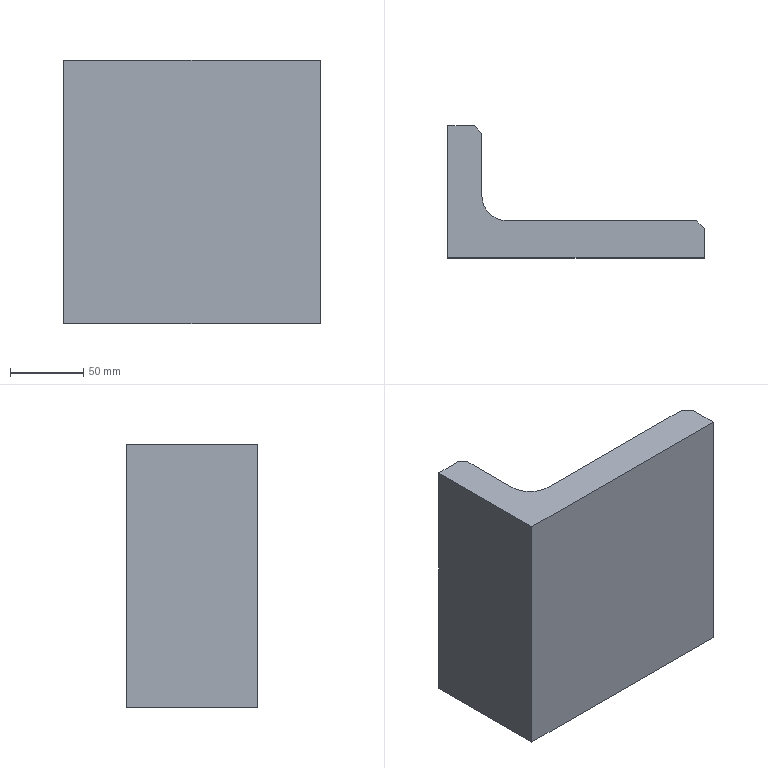Component | SolidWorks | L-Plate-1 | 1 solid | 20 faces | box 175 x 90 x 180 mm | volume 513210 mm3 | plane 18 | cylinder 2 | commonest cylinder face diameters 35.105 x2
build123d program:
from build123d import *

# Parameters (mm, degrees)
BOSS_EXTRUDE1_DEPTH = 90
BOSS_EXTRUDE3_DEPTH = 8
CHAMFER1_SIZE       = 5


with BuildPart() as part:
    # Sketch1 → Boss-Extrude1 (new, symmetric)
    with BuildSketch(Plane.XY):
        Polygon((0, 90), (0, 0), (-175, 0), (-175, 10), (-10, 10), (-10, 90), align=None)
    extrude(amount=BOSS_EXTRUDE1_DEPTH, both=True)

    # Sketch3 → Boss-Extrude3 (add)
    with BuildSketch(Plane(origin=(0, 0, -90), x_dir=(-1, 0, 0), z_dir=(0, 0, -1))):
        with BuildLine():
            Line((10, 90), (23.172, 90))
            Line((23.172, 90), (23.172, 42.657))
            ThreePointArc((23.172, 42.657), (28.312, 30.246), (40.724, 25.105))
            Line((40.724, 25.105), (175, 25.105))
            Line((175, 25.105), (175, 10))
            Line((175, 10), (10, 10))
            Line((10, 10), (10, 90))
        make_face()
    boss_extrude3 = extrude(amount=-BOSS_EXTRUDE3_DEPTH)

    # Mirror1: Boss-Extrude3 across plane
    add(boss_extrude3.mirror(Plane.XY))

    # Chamfer1
    chamfer1_edges = [part.edges().sort_by_distance(p)[0] for p in [
        (-23.172, 90, -86),
        (-175, 25.105, -86),
        (-175, 25.105, 86),
        (-23.172, 90, 86),
    ]]
    chamfer(chamfer1_edges, length=CHAMFER1_SIZE)


solid = part.part

# Placed as in the assembly
solid = solid.moved(Location((95.398, 325.813, 100), (-180, 0, 180)))
STEP:
#1=COLOUR_RGB('',0.7922,0.8196,0.9333);
#2=FILL_AREA_STYLE_COLOUR('',#1);
#3=FILL_AREA_STYLE('',(#2));
#4=SURFACE_STYLE_FILL_AREA(#3);
#5=SURFACE_SIDE_STYLE('',(#4));
#6=SURFACE_STYLE_USAGE(.BOTH.,#5);
#7=PRESENTATION_STYLE_ASSIGNMENT((#6));
#8=CARTESIAN_POINT('',(4.15,16.371,0.7087));
#9=VERTEX_POINT('',#8);
#10=CARTESIAN_POINT('',(4.15,13.221,0.7087));
#11=VERTEX_POINT('',#10);
#12=CARTESIAN_POINT('',(4.15,16.371,0.7087));
#13=DIRECTION('',(0.,-1.,0.));
#14=VECTOR('',#13,39.37);
#15=LINE('',#12,#14);
#16=EDGE_CURVE('',#9,#11,#15,.T.);
#17=ORIENTED_EDGE('',*,*,#16,.F.);
#18=CARTESIAN_POINT('',(4.15,16.371,7.165));
#19=VERTEX_POINT('',#18);
#20=CARTESIAN_POINT('',(4.15,16.371,0.3937));
#21=DIRECTION('',(0.,0.,1.));
#22=VECTOR('',#21,39.37);
#23=LINE('',#20,#22);
#24=EDGE_CURVE('',#9,#19,#23,.T.);
#25=ORIENTED_EDGE('',*,*,#24,.T.);
#26=CARTESIAN_POINT('',(4.15,13.221,7.165));
#27=VERTEX_POINT('',#26);
#28=CARTESIAN_POINT('',(4.15,16.371,7.165));
#29=DIRECTION('',(0.,-1.,0.));
#30=VECTOR('',#29,39.37);
#31=LINE('',#28,#30);
#32=EDGE_CURVE('',#19,#27,#31,.T.);
#33=ORIENTED_EDGE('',*,*,#32,.T.);
#34=CARTESIAN_POINT('',(4.15,13.221,0.3937));
#35=DIRECTION('',(0.,0.,1.));
#36=VECTOR('',#35,39.37);
#37=LINE('',#34,#36);
#38=EDGE_CURVE('',#11,#27,#37,.T.);
#39=ORIENTED_EDGE('',*,*,#38,.F.);
#40=EDGE_LOOP('',(#17,#25,#33,#39));
#41=FACE_OUTER_BOUND('',#40,.T.);
#42=CARTESIAN_POINT('',(4.15,13.221,0.3937));
#43=DIRECTION('',(-1.,0.,0.));
#44=DIRECTION('',(0.,1.,-0.));
#45=AXIS2_PLACEMENT_3D('',#42,#43,#44);
#46=PLANE('',#45);
#47=ADVANCED_FACE('',(#41),#46,.F.);
#48=CARTESIAN_POINT('',(10.646,13.221,0.7087));
#49=VERTEX_POINT('',#48);
#50=CARTESIAN_POINT('',(4.15,13.221,0.7087));
#51=DIRECTION('',(1.,-0.,-0.));
#52=VECTOR('',#51,39.37);
#53=LINE('',#50,#52);
#54=EDGE_CURVE('',#11,#49,#53,.T.);
#55=ORIENTED_EDGE('',*,*,#54,.F.);
#56=ORIENTED_EDGE('',*,*,#38,.T.);
#57=CARTESIAN_POINT('',(10.646,13.221,7.165));
#58=VERTEX_POINT('',#57);
#59=CARTESIAN_POINT('',(4.15,13.221,7.165));
#60=DIRECTION('',(1.,-0.,-0.));
#61=VECTOR('',#60,39.37);
#62=LINE('',#59,#61);
#63=EDGE_CURVE('',#27,#58,#62,.T.);
#64=ORIENTED_EDGE('',*,*,#63,.T.);
#65=CARTESIAN_POINT('',(10.646,13.221,0.3937));
#66=DIRECTION('',(0.,0.,1.));
#67=VECTOR('',#66,39.37);
#68=LINE('',#65,#67);
#69=EDGE_CURVE('',#49,#58,#68,.T.);
#70=ORIENTED_EDGE('',*,*,#69,.F.);
#71=EDGE_LOOP('',(#55,#56,#64,#70));
#72=FACE_OUTER_BOUND('',#71,.T.);
#73=CARTESIAN_POINT('',(10.646,13.221,0.3937));
#74=DIRECTION('',(-0.,-1.,0.));
#75=DIRECTION('',(-1.,0.,0.));
#76=AXIS2_PLACEMENT_3D('',#73,#74,#75);
#77=PLANE('',#76);
#78=ADVANCED_FACE('',(#72),#77,.F.);
#79=CARTESIAN_POINT('',(4.471,16.371,0.7087));
#80=VERTEX_POINT('',#79);
#81=CARTESIAN_POINT('',(4.15,16.371,0.7087));
#82=DIRECTION('',(-1.,0.,0.));
#83=VECTOR('',#82,39.37);
#84=LINE('',#81,#83);
#85=EDGE_CURVE('',#80,#9,#84,.T.);
#86=ORIENTED_EDGE('',*,*,#85,.F.);
#87=CARTESIAN_POINT('',(4.471,16.371,0.3937));
#88=VERTEX_POINT('',#87);
#89=CARTESIAN_POINT('',(4.471,16.371,0.3937));
#90=DIRECTION('',(-0.,-0.,-1.));
#91=VECTOR('',#90,39.37);
#92=LINE('',#89,#91);
#93=EDGE_CURVE('',#80,#88,#92,.T.);
#94=ORIENTED_EDGE('',*,*,#93,.T.);
#95=CARTESIAN_POINT('',(3.756,16.371,0.3937));
#96=VERTEX_POINT('',#95);
#97=CARTESIAN_POINT('',(4.15,16.371,0.3937));
#98=DIRECTION('',(1.,-0.,0.));
#99=VECTOR('',#98,39.37);
#100=LINE('',#97,#99);
#101=EDGE_CURVE('',#96,#88,#100,.T.);
#102=ORIENTED_EDGE('',*,*,#101,.F.);
#103=CARTESIAN_POINT('',(3.756,16.371,7.48));
#104=VERTEX_POINT('',#103);
#105=CARTESIAN_POINT('',(3.756,16.371,0.3937));
#106=DIRECTION('',(0.,0.,1.));
#107=VECTOR('',#106,39.37);
#108=LINE('',#105,#107);
#109=EDGE_CURVE('',#96,#104,#108,.T.);
#110=ORIENTED_EDGE('',*,*,#109,.T.);
#111=CARTESIAN_POINT('',(4.471,16.371,7.48));
#112=VERTEX_POINT('',#111);
#113=CARTESIAN_POINT('',(4.15,16.371,7.48));
#114=DIRECTION('',(1.,-0.,0.));
#115=VECTOR('',#114,39.37);
#116=LINE('',#113,#115);
#117=EDGE_CURVE('',#104,#112,#116,.T.);
#118=ORIENTED_EDGE('',*,*,#117,.T.);
#119=CARTESIAN_POINT('',(4.471,16.371,7.165));
#120=VERTEX_POINT('',#119);
#121=CARTESIAN_POINT('',(4.471,16.371,7.165));
#122=DIRECTION('',(-0.,-0.,-1.));
#123=VECTOR('',#122,39.37);
#124=LINE('',#121,#123);
#125=EDGE_CURVE('',#112,#120,#124,.T.);
#126=ORIENTED_EDGE('',*,*,#125,.T.);
#127=CARTESIAN_POINT('',(4.15,16.371,7.165));
#128=DIRECTION('',(-1.,0.,0.));
#129=VECTOR('',#128,39.37);
#130=LINE('',#127,#129);
#131=EDGE_CURVE('',#120,#19,#130,.T.);
#132=ORIENTED_EDGE('',*,*,#131,.T.);
#133=ORIENTED_EDGE('',*,*,#24,.F.);
#134=EDGE_LOOP('',(#86,#94,#102,#110,#118,#126,#132,#133));
#135=FACE_OUTER_BOUND('',#134,.T.);
#136=CARTESIAN_POINT('',(4.15,16.371,0.3937));
#137=DIRECTION('',(-0.,-1.,0.));
#138=DIRECTION('',(0.,0.,1.));
#139=AXIS2_PLACEMENT_3D('',#136,#137,#138);
#140=PLANE('',#139);
#141=ADVANCED_FACE('',(#135),#140,.F.);
#142=CARTESIAN_POINT('',(10.646,13.619,7.165));
#143=VERTEX_POINT('',#142);
#144=CARTESIAN_POINT('',(10.646,13.221,7.165));
#145=DIRECTION('',(0.,1.,-0.));
#146=VECTOR('',#145,39.37);
#147=LINE('',#144,#146);
#148=EDGE_CURVE('',#58,#143,#147,.T.);
#149=ORIENTED_EDGE('',*,*,#148,.T.);
#150=CARTESIAN_POINT('',(10.646,13.619,7.48));
#151=VERTEX_POINT('',#150);
#152=CARTESIAN_POINT('',(10.646,13.619,7.48));
#153=DIRECTION('',(0.,0.,1.));
#154=VECTOR('',#153,39.37);
#155=LINE('',#152,#154);
#156=EDGE_CURVE('',#143,#151,#155,.T.);
#157=ORIENTED_EDGE('',*,*,#156,.T.);
#158=CARTESIAN_POINT('',(10.646,12.827,7.48));
#159=VERTEX_POINT('',#158);
#160=CARTESIAN_POINT('',(10.646,12.827,7.48));
#161=DIRECTION('',(-0.,-1.,0.));
#162=VECTOR('',#161,39.37);
#163=LINE('',#160,#162);
#164=EDGE_CURVE('',#151,#159,#163,.T.);
#165=ORIENTED_EDGE('',*,*,#164,.T.);
#166=CARTESIAN_POINT('',(10.646,12.827,0.3937));
#167=VERTEX_POINT('',#166);
#168=CARTESIAN_POINT('',(10.646,12.827,0.3937));
#169=DIRECTION('',(0.,0.,1.));
#170=VECTOR('',#169,39.37);
#171=LINE('',#168,#170);
#172=EDGE_CURVE('',#167,#159,#171,.T.);
#173=ORIENTED_EDGE('',*,*,#172,.F.);
#174=CARTESIAN_POINT('',(10.646,13.619,0.3937));
#175=VERTEX_POINT('',#174);
#176=CARTESIAN_POINT('',(10.646,12.827,0.3937));
#177=DIRECTION('',(-0.,-1.,0.));
#178=VECTOR('',#177,39.37);
#179=LINE('',#176,#178);
#180=EDGE_CURVE('',#175,#167,#179,.T.);
#181=ORIENTED_EDGE('',*,*,#180,.F.);
#182=CARTESIAN_POINT('',(10.646,13.619,0.7087));
#183=VERTEX_POINT('',#182);
#184=CARTESIAN_POINT('',(10.646,13.619,0.3937));
#185=DIRECTION('',(0.,0.,1.));
#186=VECTOR('',#185,39.37);
#187=LINE('',#184,#186);
#188=EDGE_CURVE('',#175,#183,#187,.T.);
#189=ORIENTED_EDGE('',*,*,#188,.T.);
#190=CARTESIAN_POINT('',(10.646,13.221,0.7087));
#191=DIRECTION('',(0.,1.,-0.));
#192=VECTOR('',#191,39.37);
#193=LINE('',#190,#192);
#194=EDGE_CURVE('',#49,#183,#193,.T.);
#195=ORIENTED_EDGE('',*,*,#194,.F.);
#196=ORIENTED_EDGE('',*,*,#69,.T.);
#197=EDGE_LOOP('',(#149,#157,#165,#173,#181,#189,#195,#196));
#198=FACE_OUTER_BOUND('',#197,.T.);
#199=CARTESIAN_POINT('',(10.646,12.827,0.3937));
#200=DIRECTION('',(-1.,0.,0.));
#201=DIRECTION('',(0.,0.,1.));
#202=AXIS2_PLACEMENT_3D('',#199,#200,#201);
#203=PLANE('',#202);
#204=ADVANCED_FACE('',(#198),#203,.F.);
#205=CARTESIAN_POINT('',(3.756,12.827,7.48));
#206=VERTEX_POINT('',#205);
#207=CARTESIAN_POINT('',(3.756,12.827,7.48));
#208=DIRECTION('',(-1.,0.,-0.));
#209=VECTOR('',#208,39.37);
#210=LINE('',#207,#209);
#211=EDGE_CURVE('',#159,#206,#210,.T.);
#212=ORIENTED_EDGE('',*,*,#211,.T.);
#213=CARTESIAN_POINT('',(3.756,12.827,0.3937));
#214=VERTEX_POINT('',#213);
#215=CARTESIAN_POINT('',(3.756,12.827,0.3937));
#216=DIRECTION('',(0.,0.,1.));
#217=VECTOR('',#216,39.37);
#218=LINE('',#215,#217);
#219=EDGE_CURVE('',#214,#206,#218,.T.);
#220=ORIENTED_EDGE('',*,*,#219,.F.);
#221=CARTESIAN_POINT('',(3.756,12.827,0.3937));
#222=DIRECTION('',(-1.,0.,-0.));
#223=VECTOR('',#222,39.37);
#224=LINE('',#221,#223);
#225=EDGE_CURVE('',#167,#214,#224,.T.);
#226=ORIENTED_EDGE('',*,*,#225,.F.);
#227=ORIENTED_EDGE('',*,*,#172,.T.);
#228=EDGE_LOOP('',(#212,#220,#226,#227));
#229=FACE_OUTER_BOUND('',#228,.T.);
#230=CARTESIAN_POINT('',(3.756,12.827,0.3937));
#231=DIRECTION('',(0.,1.,-0.));
#232=DIRECTION('',(1.,-0.,0.));
#233=AXIS2_PLACEMENT_3D('',#230,#231,#232);
#234=PLANE('',#233);
#235=ADVANCED_FACE('',(#229),#234,.F.);
#236=CARTESIAN_POINT('',(3.756,16.371,7.48));
#237=DIRECTION('',(0.,1.,-0.));
#238=VECTOR('',#237,39.37);
#239=LINE('',#236,#238);
#240=EDGE_CURVE('',#206,#104,#239,.T.);
#241=ORIENTED_EDGE('',*,*,#240,.T.);
#242=ORIENTED_EDGE('',*,*,#109,.F.);
#243=CARTESIAN_POINT('',(3.756,16.371,0.3937));
#244=DIRECTION('',(0.,1.,-0.));
#245=VECTOR('',#244,39.37);
#246=LINE('',#243,#245);
#247=EDGE_CURVE('',#214,#96,#246,.T.);
#248=ORIENTED_EDGE('',*,*,#247,.F.);
#249=ORIENTED_EDGE('',*,*,#219,.T.);
#250=EDGE_LOOP('',(#241,#242,#248,#249));
#251=FACE_OUTER_BOUND('',#250,.T.);
#252=CARTESIAN_POINT('',(3.756,16.371,0.3937));
#253=DIRECTION('',(1.,-0.,-0.));
#254=DIRECTION('',(-0.,-1.,0.));
#255=AXIS2_PLACEMENT_3D('',#252,#253,#254);
#256=PLANE('',#255);
#257=ADVANCED_FACE('',(#251),#256,.F.);
#258=ORIENTED_EDGE('',*,*,#101,.T.);
#259=CARTESIAN_POINT('',(4.668,16.174,0.3937));
#260=VERTEX_POINT('',#259);
#261=CARTESIAN_POINT('',(4.471,16.371,0.3937));
#262=DIRECTION('',(0.7071,-0.7071,0.));
#263=VECTOR('',#262,39.37);
#264=LINE('',#261,#263);
#265=EDGE_CURVE('',#88,#260,#264,.T.);
#266=ORIENTED_EDGE('',*,*,#265,.T.);
#267=CARTESIAN_POINT('',(4.668,14.507,0.3937));
#268=VERTEX_POINT('',#267);
#269=CARTESIAN_POINT('',(4.668,16.371,0.3937));
#270=DIRECTION('',(0.,1.,-0.));
#271=VECTOR('',#270,39.37);
#272=LINE('',#269,#271);
#273=EDGE_CURVE('',#268,#260,#272,.T.);
#274=ORIENTED_EDGE('',*,*,#273,.F.);
#275=CARTESIAN_POINT('',(5.359,13.816,0.3937));
#276=VERTEX_POINT('',#275);
#277=CARTESIAN_POINT('',(5.359,14.507,0.3937));
#278=DIRECTION('',(-0.,-0.,-1.));
#279=DIRECTION('',(1.,0.,0.));
#280=AXIS2_PLACEMENT_3D('',#277,#278,#279);
#281=CIRCLE('',#280,0.691);
#282=EDGE_CURVE('',#276,#268,#281,.T.);
#283=ORIENTED_EDGE('',*,*,#282,.F.);
#284=CARTESIAN_POINT('',(10.449,13.816,0.3937));
#285=VERTEX_POINT('',#284);
#286=CARTESIAN_POINT('',(10.646,13.816,0.3937));
#287=DIRECTION('',(-1.,0.,0.));
#288=VECTOR('',#287,39.37);
#289=LINE('',#286,#288);
#290=EDGE_CURVE('',#285,#276,#289,.T.);
#291=ORIENTED_EDGE('',*,*,#290,.F.);
#292=CARTESIAN_POINT('',(10.449,13.816,0.3937));
#293=DIRECTION('',(0.7071,-0.7071,0.));
#294=VECTOR('',#293,39.37);
#295=LINE('',#292,#294);
#296=EDGE_CURVE('',#285,#175,#295,.T.);
#297=ORIENTED_EDGE('',*,*,#296,.T.);
#298=ORIENTED_EDGE('',*,*,#180,.T.);
#299=ORIENTED_EDGE('',*,*,#225,.T.);
#300=ORIENTED_EDGE('',*,*,#247,.T.);
#301=EDGE_LOOP('',(#258,#266,#274,#283,#291,#297,#298,#299,#300));
#302=FACE_OUTER_BOUND('',#301,.T.);
#303=CARTESIAN_POINT('',(3.756,12.827,0.3937));
#304=DIRECTION('',(0.,0.,1.));
#305=DIRECTION('',(1.,-0.,0.));
#306=AXIS2_PLACEMENT_3D('',#303,#304,#305);
#307=PLANE('',#306);
#308=ADVANCED_FACE('',(#302),#307,.F.);
#309=CARTESIAN_POINT('',(4.668,14.507,7.48));
#310=VERTEX_POINT('',#309);
#311=CARTESIAN_POINT('',(4.668,16.174,7.48));
#312=VERTEX_POINT('',#311);
#313=CARTESIAN_POINT('',(4.668,16.371,7.48));
#314=DIRECTION('',(0.,1.,-0.));
#315=VECTOR('',#314,39.37);
#316=LINE('',#313,#315);
#317=EDGE_CURVE('',#310,#312,#316,.T.);
#318=ORIENTED_EDGE('',*,*,#317,.T.);
#319=CARTESIAN_POINT('',(5.885,14.957,7.48));
#320=DIRECTION('',(-0.7071,0.7071,-0.));
#321=VECTOR('',#320,39.37);
#322=LINE('',#319,#321);
#323=EDGE_CURVE('',#312,#112,#322,.T.);
#324=ORIENTED_EDGE('',*,*,#323,.T.);
#325=ORIENTED_EDGE('',*,*,#117,.F.);
#326=ORIENTED_EDGE('',*,*,#240,.F.);
#327=ORIENTED_EDGE('',*,*,#211,.F.);
#328=ORIENTED_EDGE('',*,*,#164,.F.);
#329=CARTESIAN_POINT('',(10.449,13.816,7.48));
#330=VERTEX_POINT('',#329);
#331=CARTESIAN_POINT('',(7.596,16.668,7.48));
#332=DIRECTION('',(-0.7071,0.7071,-0.));
#333=VECTOR('',#332,39.37);
#334=LINE('',#331,#333);
#335=EDGE_CURVE('',#151,#330,#334,.T.);
#336=ORIENTED_EDGE('',*,*,#335,.T.);
#337=CARTESIAN_POINT('',(5.359,13.816,7.48));
#338=VERTEX_POINT('',#337);
#339=CARTESIAN_POINT('',(10.646,13.816,7.48));
#340=DIRECTION('',(-1.,0.,0.));
#341=VECTOR('',#340,39.37);
#342=LINE('',#339,#341);
#343=EDGE_CURVE('',#330,#338,#342,.T.);
#344=ORIENTED_EDGE('',*,*,#343,.T.);
#345=CARTESIAN_POINT('',(5.359,14.507,7.48));
#346=DIRECTION('',(-0.,-0.,-1.));
#347=DIRECTION('',(1.,0.,0.));
#348=AXIS2_PLACEMENT_3D('',#345,#346,#347);
#349=CIRCLE('',#348,0.691);
#350=EDGE_CURVE('',#338,#310,#349,.T.);
#351=ORIENTED_EDGE('',*,*,#350,.T.);
#352=EDGE_LOOP('',(#318,#324,#325,#326,#327,#328,#336,#344,#351));
#353=FACE_OUTER_BOUND('',#352,.T.);
#354=CARTESIAN_POINT('',(3.756,12.827,7.48));
#355=DIRECTION('',(0.,0.,1.));
#356=DIRECTION('',(1.,-0.,0.));
#357=AXIS2_PLACEMENT_3D('',#354,#355,#356);
#358=PLANE('',#357);
#359=ADVANCED_FACE('',(#353),#358,.T.);
#360=CARTESIAN_POINT('',(4.668,14.507,7.165));
#361=VERTEX_POINT('',#360);
#362=CARTESIAN_POINT('',(4.668,16.174,7.165));
#363=VERTEX_POINT('',#362);
#364=CARTESIAN_POINT('',(4.668,16.371,7.165));
#365=DIRECTION('',(0.,1.,-0.));
#366=VECTOR('',#365,39.37);
#367=LINE('',#364,#366);
#368=EDGE_CURVE('',#361,#363,#367,.T.);
#369=ORIENTED_EDGE('',*,*,#368,.T.);
#370=CARTESIAN_POINT('',(4.668,16.174,7.48));
#371=DIRECTION('',(0.,0.,1.));
#372=VECTOR('',#371,39.37);
#373=LINE('',#370,#372);
#374=EDGE_CURVE('',#363,#312,#373,.T.);
#375=ORIENTED_EDGE('',*,*,#374,.T.);
#376=ORIENTED_EDGE('',*,*,#317,.F.);
#377=CARTESIAN_POINT('',(4.668,14.507,7.165));
#378=DIRECTION('',(0.,0.,1.));
#379=VECTOR('',#378,39.37);
#380=LINE('',#377,#379);
#381=EDGE_CURVE('',#361,#310,#380,.T.);
#382=ORIENTED_EDGE('',*,*,#381,.F.);
#383=EDGE_LOOP('',(#369,#375,#376,#382));
#384=FACE_OUTER_BOUND('',#383,.T.);
#385=CARTESIAN_POINT('',(4.668,16.371,7.165));
#386=DIRECTION('',(1.,-0.,-0.));
#387=DIRECTION('',(-0.,-1.,0.));
#388=AXIS2_PLACEMENT_3D('',#385,#386,#387);
#389=PLANE('',#388);
#390=ADVANCED_FACE('',(#384),#389,.T.);
#391=ORIENTED_EDGE('',*,*,#350,.F.);
#392=CARTESIAN_POINT('',(5.359,13.816,7.165));
#393=VERTEX_POINT('',#392);
#394=CARTESIAN_POINT('',(5.359,13.816,7.165));
#395=DIRECTION('',(0.,0.,1.));
#396=VECTOR('',#395,39.37);
#397=LINE('',#394,#396);
#398=EDGE_CURVE('',#393,#338,#397,.T.);
#399=ORIENTED_EDGE('',*,*,#398,.F.);
#400=CARTESIAN_POINT('',(5.359,14.507,7.165));
#401=DIRECTION('',(-0.,-0.,-1.));
#402=DIRECTION('',(1.,0.,0.));
#403=AXIS2_PLACEMENT_3D('',#400,#401,#402);
#404=CIRCLE('',#403,0.691);
#405=EDGE_CURVE('',#393,#361,#404,.T.);
#406=ORIENTED_EDGE('',*,*,#405,.T.);
#407=ORIENTED_EDGE('',*,*,#381,.T.);
#408=EDGE_LOOP('',(#391,#399,#406,#407));
#409=FACE_OUTER_BOUND('',#408,.T.);
#410=CARTESIAN_POINT('',(5.359,14.507,7.165));
#411=DIRECTION('',(0.,0.,1.));
#412=DIRECTION('',(1.,0.,0.));
#413=AXIS2_PLACEMENT_3D('',#410,#411,#412);
#414=CYLINDRICAL_SURFACE('',#413,0.691);
#415=ADVANCED_FACE('',(#409),#414,.F.);
#416=ORIENTED_EDGE('',*,*,#343,.F.);
#417=CARTESIAN_POINT('',(10.449,13.816,7.165));
#418=VERTEX_POINT('',#417);
#419=CARTESIAN_POINT('',(10.449,13.816,7.165));
#420=DIRECTION('',(-0.,-0.,-1.));
#421=VECTOR('',#420,39.37);
#422=LINE('',#419,#421);
#423=EDGE_CURVE('',#330,#418,#422,.T.);
#424=ORIENTED_EDGE('',*,*,#423,.T.);
#425=CARTESIAN_POINT('',(10.646,13.816,7.165));
#426=DIRECTION('',(-1.,0.,0.));
#427=VECTOR('',#426,39.37);
#428=LINE('',#425,#427);
#429=EDGE_CURVE('',#418,#393,#428,.T.);
#430=ORIENTED_EDGE('',*,*,#429,.T.);
#431=ORIENTED_EDGE('',*,*,#398,.T.);
#432=EDGE_LOOP('',(#416,#424,#430,#431));
#433=FACE_OUTER_BOUND('',#432,.T.);
#434=CARTESIAN_POINT('',(10.646,13.816,7.165));
#435=DIRECTION('',(0.,1.,-0.));
#436=DIRECTION('',(1.,-0.,-0.));
#437=AXIS2_PLACEMENT_3D('',#434,#435,#436);
#438=PLANE('',#437);
#439=ADVANCED_FACE('',(#433),#438,.T.);
#440=ORIENTED_EDGE('',*,*,#131,.F.);
#441=CARTESIAN_POINT('',(4.668,16.174,7.165));
#442=DIRECTION('',(0.7071,-0.7071,0.));
#443=VECTOR('',#442,39.37);
#444=LINE('',#441,#443);
#445=EDGE_CURVE('',#120,#363,#444,.T.);
#446=ORIENTED_EDGE('',*,*,#445,.T.);
#447=ORIENTED_EDGE('',*,*,#368,.F.);
#448=ORIENTED_EDGE('',*,*,#405,.F.);
#449=ORIENTED_EDGE('',*,*,#429,.F.);
#450=CARTESIAN_POINT('',(10.646,13.619,7.165));
#451=DIRECTION('',(0.7071,-0.7071,0.));
#452=VECTOR('',#451,39.37);
#453=LINE('',#450,#452);
#454=EDGE_CURVE('',#418,#143,#453,.T.);
#455=ORIENTED_EDGE('',*,*,#454,.T.);
#456=ORIENTED_EDGE('',*,*,#148,.F.);
#457=ORIENTED_EDGE('',*,*,#63,.F.);
#458=ORIENTED_EDGE('',*,*,#32,.F.);
#459=EDGE_LOOP('',(#440,#446,#447,#448,#449,#455,#456,#457,#458));
#460=FACE_OUTER_BOUND('',#459,.T.);
#461=CARTESIAN_POINT('',(5.359,14.507,7.165));
#462=DIRECTION('',(0.,0.,1.));
#463=DIRECTION('',(1.,-0.,0.));
#464=AXIS2_PLACEMENT_3D('',#461,#462,#463);
#465=PLANE('',#464);
#466=ADVANCED_FACE('',(#460),#465,.F.);
#467=CARTESIAN_POINT('',(10.449,13.816,0.7087));
#468=VERTEX_POINT('',#467);
#469=CARTESIAN_POINT('',(5.359,13.816,0.7087));
#470=VERTEX_POINT('',#469);
#471=CARTESIAN_POINT('',(10.646,13.816,0.7087));
#472=DIRECTION('',(-1.,0.,0.));
#473=VECTOR('',#472,39.37);
#474=LINE('',#471,#473);
#475=EDGE_CURVE('',#468,#470,#474,.T.);
#476=ORIENTED_EDGE('',*,*,#475,.F.);
#477=CARTESIAN_POINT('',(10.449,13.816,0.7087));
#478=DIRECTION('',(-0.,-0.,-1.));
#479=VECTOR('',#478,39.37);
#480=LINE('',#477,#479);
#481=EDGE_CURVE('',#468,#285,#480,.T.);
#482=ORIENTED_EDGE('',*,*,#481,.T.);
#483=ORIENTED_EDGE('',*,*,#290,.T.);
#484=CARTESIAN_POINT('',(5.359,13.816,0.7087));
#485=DIRECTION('',(-0.,-0.,-1.));
#486=VECTOR('',#485,39.37);
#487=LINE('',#484,#486);
#488=EDGE_CURVE('',#470,#276,#487,.T.);
#489=ORIENTED_EDGE('',*,*,#488,.F.);
#490=EDGE_LOOP('',(#476,#482,#483,#489));
#491=FACE_OUTER_BOUND('',#490,.T.);
#492=CARTESIAN_POINT('',(10.646,13.816,0.7087));
#493=DIRECTION('',(-0.,-1.,0.));
#494=DIRECTION('',(-1.,0.,0.));
#495=AXIS2_PLACEMENT_3D('',#492,#493,#494);
#496=PLANE('',#495);
#497=ADVANCED_FACE('',(#491),#496,.F.);
#498=ORIENTED_EDGE('',*,*,#282,.T.);
#499=CARTESIAN_POINT('',(4.668,14.507,0.7087));
#500=VERTEX_POINT('',#499);
#501=CARTESIAN_POINT('',(4.668,14.507,0.7087));
#502=DIRECTION('',(-0.,-0.,-1.));
#503=VECTOR('',#502,39.37);
#504=LINE('',#501,#503);
#505=EDGE_CURVE('',#500,#268,#504,.T.);
#506=ORIENTED_EDGE('',*,*,#505,.F.);
#507=CARTESIAN_POINT('',(5.359,14.507,0.7087));
#508=DIRECTION('',(-0.,-0.,-1.));
#509=DIRECTION('',(1.,0.,0.));
#510=AXIS2_PLACEMENT_3D('',#507,#508,#509);
#511=CIRCLE('',#510,0.691);
#512=EDGE_CURVE('',#470,#500,#511,.T.);
#513=ORIENTED_EDGE('',*,*,#512,.F.);
#514=ORIENTED_EDGE('',*,*,#488,.T.);
#515=EDGE_LOOP('',(#498,#506,#513,#514));
#516=FACE_OUTER_BOUND('',#515,.T.);
#517=CARTESIAN_POINT('',(5.359,14.507,0.7087));
#518=DIRECTION('',(-0.,-0.,-1.));
#519=DIRECTION('',(-1.,0.,0.));
#520=AXIS2_PLACEMENT_3D('',#517,#518,#519);
#521=CYLINDRICAL_SURFACE('',#520,0.691);
#522=ADVANCED_FACE('',(#516),#521,.F.);
#523=ORIENTED_EDGE('',*,*,#273,.T.);
#524=CARTESIAN_POINT('',(4.668,16.174,0.7087));
#525=VERTEX_POINT('',#524);
#526=CARTESIAN_POINT('',(4.668,16.174,0.7087));
#527=DIRECTION('',(0.,0.,1.));
#528=VECTOR('',#527,39.37);
#529=LINE('',#526,#528);
#530=EDGE_CURVE('',#260,#525,#529,.T.);
#531=ORIENTED_EDGE('',*,*,#530,.T.);
#532=CARTESIAN_POINT('',(4.668,16.371,0.7087));
#533=DIRECTION('',(0.,1.,-0.));
#534=VECTOR('',#533,39.37);
#535=LINE('',#532,#534);
#536=EDGE_CURVE('',#500,#525,#535,.T.);
#537=ORIENTED_EDGE('',*,*,#536,.F.);
#538=ORIENTED_EDGE('',*,*,#505,.T.);
#539=EDGE_LOOP('',(#523,#531,#537,#538));
#540=FACE_OUTER_BOUND('',#539,.T.);
#541=CARTESIAN_POINT('',(4.668,16.371,0.7087));
#542=DIRECTION('',(-1.,0.,0.));
#543=DIRECTION('',(0.,1.,-0.));
#544=AXIS2_PLACEMENT_3D('',#541,#542,#543);
#545=PLANE('',#544);
#546=ADVANCED_FACE('',(#540),#545,.F.);
#547=ORIENTED_EDGE('',*,*,#536,.T.);
#548=CARTESIAN_POINT('',(4.471,16.371,0.7087));
#549=DIRECTION('',(-0.7071,0.7071,-0.));
#550=VECTOR('',#549,39.37);
#551=LINE('',#548,#550);
#552=EDGE_CURVE('',#525,#80,#551,.T.);
#553=ORIENTED_EDGE('',*,*,#552,.T.);
#554=ORIENTED_EDGE('',*,*,#85,.T.);
#555=ORIENTED_EDGE('',*,*,#16,.T.);
#556=ORIENTED_EDGE('',*,*,#54,.T.);
#557=ORIENTED_EDGE('',*,*,#194,.T.);
#558=CARTESIAN_POINT('',(10.449,13.816,0.7087));
#559=DIRECTION('',(-0.7071,0.7071,-0.));
#560=VECTOR('',#559,39.37);
#561=LINE('',#558,#560);
#562=EDGE_CURVE('',#183,#468,#561,.T.);
#563=ORIENTED_EDGE('',*,*,#562,.T.);
#564=ORIENTED_EDGE('',*,*,#475,.T.);
#565=ORIENTED_EDGE('',*,*,#512,.T.);
#566=EDGE_LOOP('',(#547,#553,#554,#555,#556,#557,#563,#564,#565));
#567=FACE_OUTER_BOUND('',#566,.T.);
#568=CARTESIAN_POINT('',(5.359,14.507,0.7087));
#569=DIRECTION('',(-0.,-0.,-1.));
#570=DIRECTION('',(1.,-0.,0.));
#571=AXIS2_PLACEMENT_3D('',#568,#569,#570);
#572=PLANE('',#571);
#573=ADVANCED_FACE('',(#567),#572,.F.);
#574=ORIENTED_EDGE('',*,*,#552,.F.);
#575=ORIENTED_EDGE('',*,*,#530,.F.);
#576=ORIENTED_EDGE('',*,*,#265,.F.);
#577=ORIENTED_EDGE('',*,*,#93,.F.);
#578=EDGE_LOOP('',(#574,#575,#576,#577));
#579=FACE_OUTER_BOUND('',#578,.T.);
#580=CARTESIAN_POINT('',(4.471,16.371,0.3937));
#581=DIRECTION('',(-0.7071,-0.7071,0.));
#582=DIRECTION('',(-0.,-0.,-1.));
#583=AXIS2_PLACEMENT_3D('',#580,#581,#582);
#584=PLANE('',#583);
#585=ADVANCED_FACE('',(#579),#584,.F.);
#586=ORIENTED_EDGE('',*,*,#445,.F.);
#587=ORIENTED_EDGE('',*,*,#125,.F.);
#588=ORIENTED_EDGE('',*,*,#323,.F.);
#589=ORIENTED_EDGE('',*,*,#374,.F.);
#590=EDGE_LOOP('',(#586,#587,#588,#589));
#591=FACE_OUTER_BOUND('',#590,.T.);
#592=CARTESIAN_POINT('',(4.668,16.174,7.165));
#593=DIRECTION('',(0.7071,0.7071,-0.));
#594=DIRECTION('',(-0.,-0.,-1.));
#595=AXIS2_PLACEMENT_3D('',#592,#593,#594);
#596=PLANE('',#595);
#597=ADVANCED_FACE('',(#591),#596,.T.);
#598=ORIENTED_EDGE('',*,*,#454,.F.);
#599=ORIENTED_EDGE('',*,*,#423,.F.);
#600=ORIENTED_EDGE('',*,*,#335,.F.);
#601=ORIENTED_EDGE('',*,*,#156,.F.);
#602=EDGE_LOOP('',(#598,#599,#600,#601));
#603=FACE_OUTER_BOUND('',#602,.T.);
#604=CARTESIAN_POINT('',(10.646,13.619,0.3937));
#605=DIRECTION('',(0.7071,0.7071,-0.));
#606=DIRECTION('',(-0.,-0.,-1.));
#607=AXIS2_PLACEMENT_3D('',#604,#605,#606);
#608=PLANE('',#607);
#609=ADVANCED_FACE('',(#603),#608,.T.);
#610=ORIENTED_EDGE('',*,*,#562,.F.);
#611=ORIENTED_EDGE('',*,*,#188,.F.);
#612=ORIENTED_EDGE('',*,*,#296,.F.);
#613=ORIENTED_EDGE('',*,*,#481,.F.);
#614=EDGE_LOOP('',(#610,#611,#612,#613));
#615=FACE_OUTER_BOUND('',#614,.T.);
#616=CARTESIAN_POINT('',(10.449,13.816,0.7087));
#617=DIRECTION('',(-0.7071,-0.7071,0.));
#618=DIRECTION('',(-0.,-0.,-1.));
#619=AXIS2_PLACEMENT_3D('',#616,#617,#618);
#620=PLANE('',#619);
#621=ADVANCED_FACE('',(#615),#620,.F.);
#622=CLOSED_SHELL('',(#47,#78,#141,#204,#235,#257,#308,#359,#390,#415,#439,#466,#497,#522,#546,#573,#585,#597,#609,#621));
#623=MANIFOLD_SOLID_BREP('',#622);
#624=STYLED_ITEM('',(#7),#623);
#625=(LENGTH_UNIT()NAMED_UNIT(*)SI_UNIT($,.METRE.));
#626=LENGTH_MEASURE_WITH_UNIT(LENGTH_MEASURE(0.0254),#625);
#627=DIMENSIONAL_EXPONENTS(1.,0.,0.,0.,0.,0.,0.);
#628=(CONVERSION_BASED_UNIT('',#626)LENGTH_UNIT()NAMED_UNIT(#627));
#629=UNCERTAINTY_MEASURE_WITH_UNIT(LENGTH_MEASURE(0.00001),#628,'','');
#630=(NAMED_UNIT(*)PLANE_ANGLE_UNIT()SI_UNIT($,.RADIAN.));
#631=(NAMED_UNIT(*)SI_UNIT($,.STERADIAN.)SOLID_ANGLE_UNIT());
#632=(GEOMETRIC_REPRESENTATION_CONTEXT(3)GLOBAL_UNCERTAINTY_ASSIGNED_CONTEXT((#629))GLOBAL_UNIT_ASSIGNED_CONTEXT((#628,#630,#631))REPRESENTATION_CONTEXT('',''));
#633=MECHANICAL_DESIGN_GEOMETRIC_PRESENTATION_REPRESENTATION('',(#624),#632);
#634=CARTESIAN_POINT('',(0.,0.,0.));
#635=DIRECTION('',(0.,0.,1.));
#636=DIRECTION('',(1.,0.,0.));
#637=AXIS2_PLACEMENT_3D('',#634,#635,#636);
#638=(LENGTH_UNIT()NAMED_UNIT(*)SI_UNIT($,.METRE.));
#639=LENGTH_MEASURE_WITH_UNIT(LENGTH_MEASURE(0.0254),#638);
#640=DIMENSIONAL_EXPONENTS(1.,0.,0.,0.,0.,0.,0.);
#641=(CONVERSION_BASED_UNIT('',#639)LENGTH_UNIT()NAMED_UNIT(#640));
#642=UNCERTAINTY_MEASURE_WITH_UNIT(LENGTH_MEASURE(0.00001),#641,'','');
#643=(NAMED_UNIT(*)PLANE_ANGLE_UNIT()SI_UNIT($,.RADIAN.));
#644=(NAMED_UNIT(*)SI_UNIT($,.STERADIAN.)SOLID_ANGLE_UNIT());
#645=(GEOMETRIC_REPRESENTATION_CONTEXT(3)GLOBAL_UNCERTAINTY_ASSIGNED_CONTEXT((#642))GLOBAL_UNIT_ASSIGNED_CONTEXT((#641,#643,#644))REPRESENTATION_CONTEXT('',''));
#646=ADVANCED_BREP_SHAPE_REPRESENTATION('',(#623,#637),#645);
#647=PRESENTATION_LAYER_ASSIGNMENT('','',(#624));